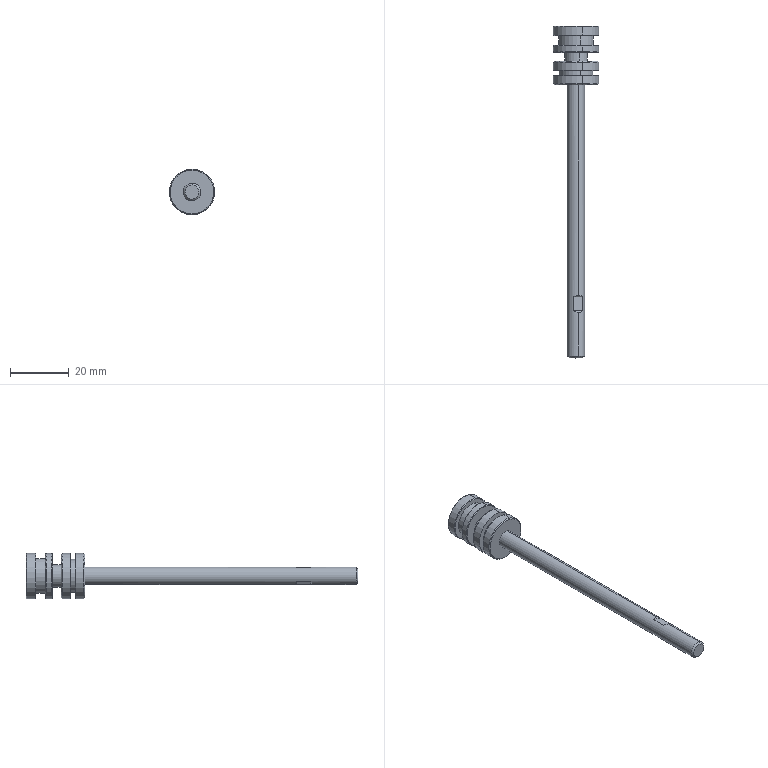Component | SolidWorks | gbgbMA16x35SCA_0_+-2_gbgb2-1 | 1 solid | 45 faces | volume 5544 mm3 | cylinder 16 | plane 15 | cone 14 | commonest cylinder face diameters 15.5 x8 6 x2 11.4 x2 7.7 x2 11.9 x2